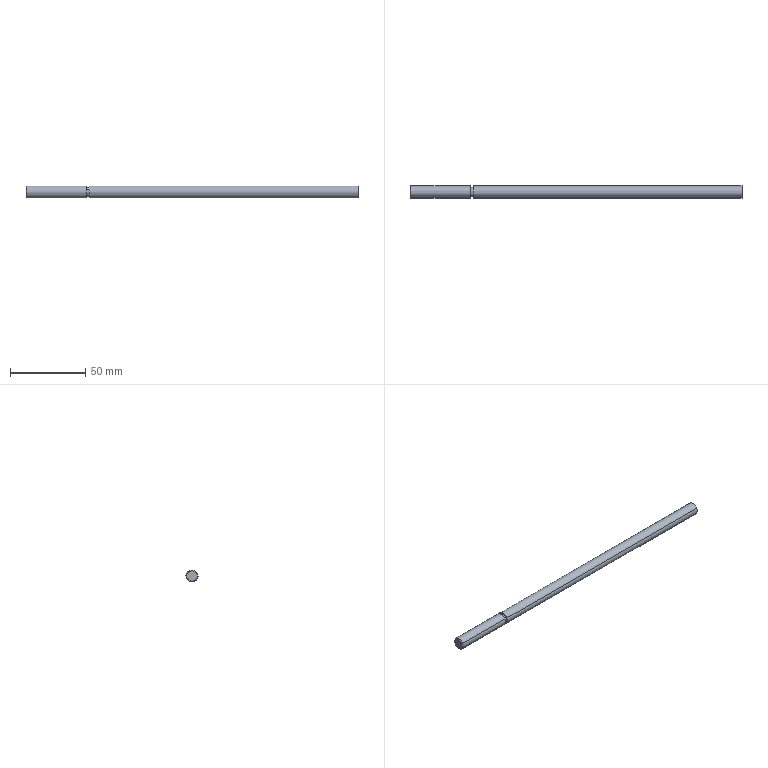Component | SolidWorks | 007GuideRod-2 | 1 solid | 16 faces | box 220 x 8 x 8 mm | volume 10834 mm3 | cylinder 8 | cone 4 | plane 4 | commonest cylinder face diameters 8 x4 6 x2 4.2 x2
build123d program:
from build123d import *

# Parameters (mm, degrees)
SKETCH1_R                 = 4
EXTRUDE1_DEPTH            = 110
M5X0_8_TAPPED_HOLE1_D     = 4.2
M5X0_8_TAPPED_HOLE1_DEPTH = 12.4
M5X0_8_TAPPED_HOLE1_TIP   = 1.262
CHAMFER1_SIZE             = 0.5
SKETCH4_W                 = 1
SKETCH4_H                 = 2


with BuildPart() as part:
    # Sketch1 → Extrude1 (new, symmetric)
    with BuildSketch(Plane.XY):
        Circle(SKETCH1_R)
    extrude(amount=EXTRUDE1_DEPTH, both=True)

    # M5x0.8 Tapped Hole1
    with Locations(Plane.XY.offset(110)):
        with Locations((0, 0)):
            Hole(M5X0_8_TAPPED_HOLE1_D / 2, depth=M5X0_8_TAPPED_HOLE1_DEPTH)
            with Locations((0, 0, -(M5X0_8_TAPPED_HOLE1_DEPTH + M5X0_8_TAPPED_HOLE1_TIP / 2))):  # 118° drill point
                Cone(0, M5X0_8_TAPPED_HOLE1_D / 2, M5X0_8_TAPPED_HOLE1_TIP, mode=Mode.SUBTRACT)

    # Chamfer1
    chamfer1_edges = [part.edges().sort_by_distance(p)[0] for p in [
        (-4, 0, -110),
    ]]
    chamfer(chamfer1_edges, length=CHAMFER1_SIZE)

    # Sketch4 → Cut-Revolve1 (revolve, cut)
    with BuildSketch(Plane(origin=(0, 0, 0), x_dir=(1, 0, 0), z_dir=(0, 1, 0))):
        with Locations((-3.5, 69)):
            Rectangle(SKETCH4_W, SKETCH4_H)
    revolve(axis=Axis((0, 0, -71.443), (0, 0, 1)), mode=Mode.SUBTRACT)


solid = part.part

# Placed as in the assembly
solid = solid.moved(Location((-83.24, 24.924, 53.04), (0, 90, 0)))
STEP:
#1=CARTESIAN_POINT('',(-6.033,1.121,2.016));
#2=VERTEX_POINT('',#1);
#3=CARTESIAN_POINT('',(-6.033,0.8413,2.16));
#4=VERTEX_POINT('',#3);
#5=CARTESIAN_POINT('',(-6.033,0.9813,2.088));
#6=DIRECTION('',(-1.,-0.,0.));
#7=DIRECTION('',(0.,0.8889,-0.4581));
#8=AXIS2_PLACEMENT_3D('',#5,#6,#7);
#9=CIRCLE('',#8,0.1575);
#10=EDGE_CURVE('',#2,#4,#9,.T.);
#11=ORIENTED_EDGE('',*,*,#10,.T.);
#12=CARTESIAN_POINT('',(-7.588,0.8413,2.16));
#13=VERTEX_POINT('',#12);
#14=CARTESIAN_POINT('',(1.054,0.8413,2.16));
#15=DIRECTION('',(-1.,-0.,0.));
#16=VECTOR('',#15,39.37);
#17=LINE('',#14,#16);
#18=EDGE_CURVE('',#4,#13,#17,.T.);
#19=ORIENTED_EDGE('',*,*,#18,.T.);
#20=CARTESIAN_POINT('',(-7.588,1.121,2.016));
#21=VERTEX_POINT('',#20);
#22=CARTESIAN_POINT('',(-7.588,0.9813,2.088));
#23=DIRECTION('',(1.,0.,-0.));
#24=DIRECTION('',(0.,-0.8889,0.4581));
#25=AXIS2_PLACEMENT_3D('',#22,#23,#24);
#26=CIRCLE('',#25,0.1575);
#27=EDGE_CURVE('',#13,#21,#26,.T.);
#28=ORIENTED_EDGE('',*,*,#27,.T.);
#29=CARTESIAN_POINT('',(1.054,1.121,2.016));
#30=DIRECTION('',(-1.,-0.,0.));
#31=VECTOR('',#30,39.37);
#32=LINE('',#29,#31);
#33=EDGE_CURVE('',#2,#21,#32,.T.);
#34=ORIENTED_EDGE('',*,*,#33,.F.);
#35=EDGE_LOOP('',(#11,#19,#28,#34));
#36=FACE_OUTER_BOUND('',#35,.T.);
#37=CARTESIAN_POINT('',(1.054,0.9813,2.088));
#38=DIRECTION('',(-1.,-0.,0.));
#39=DIRECTION('',(0.,0.8889,-0.4581));
#40=AXIS2_PLACEMENT_3D('',#37,#38,#39);
#41=CYLINDRICAL_SURFACE('',#40,0.1575);
#42=ADVANCED_FACE('',(#36),#41,.T.);
#43=CARTESIAN_POINT('',(-7.608,1.104,2.025));
#44=VERTEX_POINT('',#43);
#45=CARTESIAN_POINT('',(-7.608,0.8588,2.151));
#46=VERTEX_POINT('',#45);
#47=CARTESIAN_POINT('',(-7.608,0.9813,2.088));
#48=DIRECTION('',(-1.,-0.,0.));
#49=DIRECTION('',(0.,-0.8889,0.4581));
#50=AXIS2_PLACEMENT_3D('',#47,#48,#49);
#51=CIRCLE('',#50,0.1378);
#52=EDGE_CURVE('',#44,#46,#51,.T.);
#53=ORIENTED_EDGE('',*,*,#52,.F.);
#54=CARTESIAN_POINT('',(-7.588,1.121,2.016));
#55=DIRECTION('',(0.7071,0.6285,-0.3239));
#56=VECTOR('',#55,39.37);
#57=LINE('',#54,#56);
#58=EDGE_CURVE('',#44,#21,#57,.T.);
#59=ORIENTED_EDGE('',*,*,#58,.T.);
#60=ORIENTED_EDGE('',*,*,#27,.F.);
#61=CARTESIAN_POINT('',(-7.588,0.8413,2.16));
#62=DIRECTION('',(0.7071,-0.6285,0.3239));
#63=VECTOR('',#62,39.37);
#64=LINE('',#61,#63);
#65=EDGE_CURVE('',#46,#13,#64,.T.);
#66=ORIENTED_EDGE('',*,*,#65,.F.);
#67=EDGE_LOOP('',(#53,#59,#60,#66));
#68=FACE_OUTER_BOUND('',#67,.T.);
#69=CARTESIAN_POINT('',(-7.588,0.9813,2.088));
#70=DIRECTION('',(1.,0.,-0.));
#71=DIRECTION('',(0.,-0.8889,0.4581));
#72=AXIS2_PLACEMENT_3D('',#69,#70,#71);
#73=CONICAL_SURFACE('',#72,0.1575,0.7854);
#74=ADVANCED_FACE('',(#68),#73,.T.);
#75=CARTESIAN_POINT('',(-5.954,1.086,2.034));
#76=VERTEX_POINT('',#75);
#77=CARTESIAN_POINT('',(-5.954,0.8763,2.142));
#78=VERTEX_POINT('',#77);
#79=CARTESIAN_POINT('',(-5.954,0.9813,2.088));
#80=DIRECTION('',(-1.,-0.,0.));
#81=DIRECTION('',(0.,0.8889,-0.4581));
#82=AXIS2_PLACEMENT_3D('',#79,#80,#81);
#83=CIRCLE('',#82,0.1181);
#84=EDGE_CURVE('',#76,#78,#83,.T.);
#85=ORIENTED_EDGE('',*,*,#84,.T.);
#86=CARTESIAN_POINT('',(-6.033,0.8763,2.142));
#87=VERTEX_POINT('',#86);
#88=CARTESIAN_POINT('',(-6.09,0.8763,2.142));
#89=DIRECTION('',(-1.,-0.,0.));
#90=VECTOR('',#89,39.37);
#91=LINE('',#88,#90);
#92=EDGE_CURVE('',#78,#87,#91,.T.);
#93=ORIENTED_EDGE('',*,*,#92,.T.);
#94=CARTESIAN_POINT('',(-6.033,1.086,2.034));
#95=VERTEX_POINT('',#94);
#96=CARTESIAN_POINT('',(-6.033,0.9813,2.088));
#97=DIRECTION('',(-1.,-0.,0.));
#98=DIRECTION('',(0.,0.8889,-0.4581));
#99=AXIS2_PLACEMENT_3D('',#96,#97,#98);
#100=CIRCLE('',#99,0.1181);
#101=EDGE_CURVE('',#95,#87,#100,.T.);
#102=ORIENTED_EDGE('',*,*,#101,.F.);
#103=CARTESIAN_POINT('',(-6.09,1.086,2.034));
#104=DIRECTION('',(-1.,-0.,0.));
#105=VECTOR('',#104,39.37);
#106=LINE('',#103,#105);
#107=EDGE_CURVE('',#76,#95,#106,.T.);
#108=ORIENTED_EDGE('',*,*,#107,.F.);
#109=EDGE_LOOP('',(#85,#93,#102,#108));
#110=FACE_OUTER_BOUND('',#109,.T.);
#111=CARTESIAN_POINT('',(-6.09,0.9813,2.088));
#112=DIRECTION('',(-1.,-0.,0.));
#113=DIRECTION('',(0.,0.8889,-0.4581));
#114=AXIS2_PLACEMENT_3D('',#111,#112,#113);
#115=CYLINDRICAL_SURFACE('',#114,0.1181);
#116=ADVANCED_FACE('',(#110),#115,.T.);
#117=CARTESIAN_POINT('',(0.5157,0.9813,2.088));
#118=VERTEX_POINT('',#117);
#119=CARTESIAN_POINT('',(0.5653,0.9078,2.126));
#120=VERTEX_POINT('',#119);
#121=CARTESIAN_POINT('',(0.5653,0.9078,2.126));
#122=DIRECTION('',(0.515,-0.7619,0.3927));
#123=VECTOR('',#122,39.37);
#124=LINE('',#121,#123);
#125=EDGE_CURVE('',#118,#120,#124,.T.);
#126=ORIENTED_EDGE('',*,*,#125,.F.);
#127=CARTESIAN_POINT('',(0.5653,1.055,2.05));
#128=VERTEX_POINT('',#127);
#129=CARTESIAN_POINT('',(0.5653,1.055,2.05));
#130=DIRECTION('',(0.515,0.7619,-0.3927));
#131=VECTOR('',#130,39.37);
#132=LINE('',#129,#131);
#133=EDGE_CURVE('',#118,#128,#132,.T.);
#134=ORIENTED_EDGE('',*,*,#133,.T.);
#135=CARTESIAN_POINT('',(0.5653,0.9813,2.088));
#136=DIRECTION('',(1.,0.,-0.));
#137=DIRECTION('',(0.,-0.8889,0.4581));
#138=AXIS2_PLACEMENT_3D('',#135,#136,#137);
#139=CIRCLE('',#138,0.08268);
#140=EDGE_CURVE('',#128,#120,#139,.T.);
#141=ORIENTED_EDGE('',*,*,#140,.T.);
#142=EDGE_LOOP('',(#126,#134,#141));
#143=FACE_OUTER_BOUND('',#142,.T.);
#144=CARTESIAN_POINT('',(0.5653,0.9813,2.088));
#145=DIRECTION('',(1.,0.,-0.));
#146=DIRECTION('',(0.,-0.8889,0.4581));
#147=AXIS2_PLACEMENT_3D('',#144,#145,#146);
#148=CONICAL_SURFACE('',#147,0.08268,1.03);
#149=ADVANCED_FACE('',(#143),#148,.F.);
#150=ORIENTED_EDGE('',*,*,#140,.F.);
#151=CARTESIAN_POINT('',(1.054,1.055,2.05));
#152=VERTEX_POINT('',#151);
#153=CARTESIAN_POINT('',(1.054,1.055,2.05));
#154=DIRECTION('',(1.,0.,-0.));
#155=VECTOR('',#154,39.37);
#156=LINE('',#153,#155);
#157=EDGE_CURVE('',#128,#152,#156,.T.);
#158=ORIENTED_EDGE('',*,*,#157,.T.);
#159=CARTESIAN_POINT('',(1.054,0.9078,2.126));
#160=VERTEX_POINT('',#159);
#161=CARTESIAN_POINT('',(1.054,0.9813,2.088));
#162=DIRECTION('',(1.,0.,-0.));
#163=DIRECTION('',(0.,-0.8889,0.4581));
#164=AXIS2_PLACEMENT_3D('',#161,#162,#163);
#165=CIRCLE('',#164,0.08268);
#166=EDGE_CURVE('',#152,#160,#165,.T.);
#167=ORIENTED_EDGE('',*,*,#166,.T.);
#168=CARTESIAN_POINT('',(1.054,0.9078,2.126));
#169=DIRECTION('',(1.,0.,-0.));
#170=VECTOR('',#169,39.37);
#171=LINE('',#168,#170);
#172=EDGE_CURVE('',#120,#160,#171,.T.);
#173=ORIENTED_EDGE('',*,*,#172,.F.);
#174=EDGE_LOOP('',(#150,#158,#167,#173));
#175=FACE_OUTER_BOUND('',#174,.T.);
#176=CARTESIAN_POINT('',(1.054,0.9813,2.088));
#177=DIRECTION('',(1.,0.,-0.));
#178=DIRECTION('',(0.,-0.8889,0.4581));
#179=AXIS2_PLACEMENT_3D('',#176,#177,#178);
#180=CYLINDRICAL_SURFACE('',#179,0.08268);
#181=ADVANCED_FACE('',(#175),#180,.F.);
#182=CARTESIAN_POINT('',(1.054,0.8413,2.16));
#183=VERTEX_POINT('',#182);
#184=CARTESIAN_POINT('',(1.054,1.121,2.016));
#185=VERTEX_POINT('',#184);
#186=CARTESIAN_POINT('',(1.054,0.9813,2.088));
#187=DIRECTION('',(1.,0.,-0.));
#188=DIRECTION('',(0.,-0.8889,0.4581));
#189=AXIS2_PLACEMENT_3D('',#186,#187,#188);
#190=CIRCLE('',#189,0.1575);
#191=EDGE_CURVE('',#183,#185,#190,.T.);
#192=ORIENTED_EDGE('',*,*,#191,.F.);
#193=CARTESIAN_POINT('',(-5.954,0.8413,2.16));
#194=VERTEX_POINT('',#193);
#195=CARTESIAN_POINT('',(1.054,0.8413,2.16));
#196=DIRECTION('',(-1.,-0.,0.));
#197=VECTOR('',#196,39.37);
#198=LINE('',#195,#197);
#199=EDGE_CURVE('',#183,#194,#198,.T.);
#200=ORIENTED_EDGE('',*,*,#199,.T.);
#201=CARTESIAN_POINT('',(-5.954,1.121,2.016));
#202=VERTEX_POINT('',#201);
#203=CARTESIAN_POINT('',(-5.954,0.9813,2.088));
#204=DIRECTION('',(-1.,-0.,0.));
#205=DIRECTION('',(0.,0.8889,-0.4581));
#206=AXIS2_PLACEMENT_3D('',#203,#204,#205);
#207=CIRCLE('',#206,0.1575);
#208=EDGE_CURVE('',#202,#194,#207,.T.);
#209=ORIENTED_EDGE('',*,*,#208,.F.);
#210=CARTESIAN_POINT('',(1.054,1.121,2.016));
#211=DIRECTION('',(-1.,-0.,0.));
#212=VECTOR('',#211,39.37);
#213=LINE('',#210,#212);
#214=EDGE_CURVE('',#185,#202,#213,.T.);
#215=ORIENTED_EDGE('',*,*,#214,.F.);
#216=EDGE_LOOP('',(#192,#200,#209,#215));
#217=FACE_OUTER_BOUND('',#216,.T.);
#218=CARTESIAN_POINT('',(1.054,0.9813,2.088));
#219=DIRECTION('',(-1.,-0.,0.));
#220=DIRECTION('',(0.,0.8889,-0.4581));
#221=AXIS2_PLACEMENT_3D('',#218,#219,#220);
#222=CYLINDRICAL_SURFACE('',#221,0.1575);
#223=ADVANCED_FACE('',(#217),#222,.T.);
#224=ORIENTED_EDGE('',*,*,#199,.F.);
#225=CARTESIAN_POINT('',(1.054,0.9813,2.088));
#226=DIRECTION('',(1.,0.,-0.));
#227=DIRECTION('',(0.,-0.8889,0.4581));
#228=AXIS2_PLACEMENT_3D('',#225,#226,#227);
#229=CIRCLE('',#228,0.1575);
#230=EDGE_CURVE('',#185,#183,#229,.T.);
#231=ORIENTED_EDGE('',*,*,#230,.F.);
#232=ORIENTED_EDGE('',*,*,#214,.T.);
#233=CARTESIAN_POINT('',(-5.954,0.9813,2.088));
#234=DIRECTION('',(-1.,-0.,0.));
#235=DIRECTION('',(0.,0.8889,-0.4581));
#236=AXIS2_PLACEMENT_3D('',#233,#234,#235);
#237=CIRCLE('',#236,0.1575);
#238=EDGE_CURVE('',#194,#202,#237,.T.);
#239=ORIENTED_EDGE('',*,*,#238,.F.);
#240=EDGE_LOOP('',(#224,#231,#232,#239));
#241=FACE_OUTER_BOUND('',#240,.T.);
#242=CARTESIAN_POINT('',(1.054,0.9813,2.088));
#243=DIRECTION('',(-1.,-0.,0.));
#244=DIRECTION('',(0.,0.8889,-0.4581));
#245=AXIS2_PLACEMENT_3D('',#242,#243,#244);
#246=CYLINDRICAL_SURFACE('',#245,0.1575);
#247=ADVANCED_FACE('',(#241),#246,.T.);
#248=CARTESIAN_POINT('',(1.054,0.9813,2.088));
#249=DIRECTION('',(1.,0.,-0.));
#250=DIRECTION('',(0.,-0.8889,0.4581));
#251=AXIS2_PLACEMENT_3D('',#248,#249,#250);
#252=CIRCLE('',#251,0.08268);
#253=EDGE_CURVE('',#160,#152,#252,.T.);
#254=ORIENTED_EDGE('',*,*,#253,.F.);
#255=ORIENTED_EDGE('',*,*,#166,.F.);
#256=EDGE_LOOP('',(#254,#255));
#257=FACE_BOUND('',#256,.T.);
#258=ORIENTED_EDGE('',*,*,#230,.T.);
#259=ORIENTED_EDGE('',*,*,#191,.T.);
#260=EDGE_LOOP('',(#258,#259));
#261=FACE_OUTER_BOUND('',#260,.T.);
#262=CARTESIAN_POINT('',(1.054,0.9813,2.088));
#263=DIRECTION('',(1.,0.,-0.));
#264=DIRECTION('',(0.,-0.8889,0.4581));
#265=AXIS2_PLACEMENT_3D('',#262,#263,#264);
#266=PLANE('',#265);
#267=ADVANCED_FACE('',(#257,#261),#266,.T.);
#268=ORIENTED_EDGE('',*,*,#157,.F.);
#269=CARTESIAN_POINT('',(0.5653,0.9813,2.088));
#270=DIRECTION('',(1.,0.,-0.));
#271=DIRECTION('',(0.,-0.8889,0.4581));
#272=AXIS2_PLACEMENT_3D('',#269,#270,#271);
#273=CIRCLE('',#272,0.08268);
#274=EDGE_CURVE('',#120,#128,#273,.T.);
#275=ORIENTED_EDGE('',*,*,#274,.F.);
#276=ORIENTED_EDGE('',*,*,#172,.T.);
#277=ORIENTED_EDGE('',*,*,#253,.T.);
#278=EDGE_LOOP('',(#268,#275,#276,#277));
#279=FACE_OUTER_BOUND('',#278,.T.);
#280=CARTESIAN_POINT('',(1.054,0.9813,2.088));
#281=DIRECTION('',(1.,0.,-0.));
#282=DIRECTION('',(0.,-0.8889,0.4581));
#283=AXIS2_PLACEMENT_3D('',#280,#281,#282);
#284=CYLINDRICAL_SURFACE('',#283,0.08268);
#285=ADVANCED_FACE('',(#279),#284,.F.);
#286=ORIENTED_EDGE('',*,*,#133,.F.);
#287=ORIENTED_EDGE('',*,*,#125,.T.);
#288=ORIENTED_EDGE('',*,*,#274,.T.);
#289=EDGE_LOOP('',(#286,#287,#288));
#290=FACE_OUTER_BOUND('',#289,.T.);
#291=CARTESIAN_POINT('',(0.5653,0.9813,2.088));
#292=DIRECTION('',(1.,0.,-0.));
#293=DIRECTION('',(0.,-0.8889,0.4581));
#294=AXIS2_PLACEMENT_3D('',#291,#292,#293);
#295=CONICAL_SURFACE('',#294,0.08268,1.03);
#296=ADVANCED_FACE('',(#290),#295,.F.);
#297=ORIENTED_EDGE('',*,*,#10,.F.);
#298=CARTESIAN_POINT('',(-6.033,0.9813,2.088));
#299=DIRECTION('',(-1.,-0.,0.));
#300=DIRECTION('',(0.,0.8889,-0.4581));
#301=AXIS2_PLACEMENT_3D('',#298,#299,#300);
#302=CIRCLE('',#301,0.1575);
#303=EDGE_CURVE('',#4,#2,#302,.T.);
#304=ORIENTED_EDGE('',*,*,#303,.F.);
#305=EDGE_LOOP('',(#297,#304));
#306=FACE_OUTER_BOUND('',#305,.T.);
#307=ORIENTED_EDGE('',*,*,#101,.T.);
#308=CARTESIAN_POINT('',(-6.033,0.9813,2.088));
#309=DIRECTION('',(-1.,-0.,0.));
#310=DIRECTION('',(0.,0.8889,-0.4581));
#311=AXIS2_PLACEMENT_3D('',#308,#309,#310);
#312=CIRCLE('',#311,0.1181);
#313=EDGE_CURVE('',#87,#95,#312,.T.);
#314=ORIENTED_EDGE('',*,*,#313,.T.);
#315=EDGE_LOOP('',(#307,#314));
#316=FACE_BOUND('',#315,.T.);
#317=CARTESIAN_POINT('',(-6.033,1.121,2.016));
#318=DIRECTION('',(-1.,-0.,0.));
#319=DIRECTION('',(-0.,0.8889,-0.4581));
#320=AXIS2_PLACEMENT_3D('',#317,#318,#319);
#321=PLANE('',#320);
#322=ADVANCED_FACE('',(#306,#316),#321,.F.);
#323=ORIENTED_EDGE('',*,*,#92,.F.);
#324=CARTESIAN_POINT('',(-5.954,0.9813,2.088));
#325=DIRECTION('',(-1.,-0.,0.));
#326=DIRECTION('',(0.,0.8889,-0.4581));
#327=AXIS2_PLACEMENT_3D('',#324,#325,#326);
#328=CIRCLE('',#327,0.1181);
#329=EDGE_CURVE('',#78,#76,#328,.T.);
#330=ORIENTED_EDGE('',*,*,#329,.T.);
#331=ORIENTED_EDGE('',*,*,#107,.T.);
#332=ORIENTED_EDGE('',*,*,#313,.F.);
#333=EDGE_LOOP('',(#323,#330,#331,#332));
#334=FACE_OUTER_BOUND('',#333,.T.);
#335=CARTESIAN_POINT('',(-6.09,0.9813,2.088));
#336=DIRECTION('',(-1.,-0.,0.));
#337=DIRECTION('',(0.,0.8889,-0.4581));
#338=AXIS2_PLACEMENT_3D('',#335,#336,#337);
#339=CYLINDRICAL_SURFACE('',#338,0.1181);
#340=ADVANCED_FACE('',(#334),#339,.T.);
#341=ORIENTED_EDGE('',*,*,#84,.F.);
#342=ORIENTED_EDGE('',*,*,#329,.F.);
#343=EDGE_LOOP('',(#341,#342));
#344=FACE_BOUND('',#343,.T.);
#345=ORIENTED_EDGE('',*,*,#208,.T.);
#346=ORIENTED_EDGE('',*,*,#238,.T.);
#347=EDGE_LOOP('',(#345,#346));
#348=FACE_OUTER_BOUND('',#347,.T.);
#349=CARTESIAN_POINT('',(-5.954,1.086,2.034));
#350=DIRECTION('',(1.,0.,-0.));
#351=DIRECTION('',(0.,-0.8889,0.4581));
#352=AXIS2_PLACEMENT_3D('',#349,#350,#351);
#353=PLANE('',#352);
#354=ADVANCED_FACE('',(#344,#348),#353,.F.);
#355=CARTESIAN_POINT('',(-7.608,0.9813,2.088));
#356=DIRECTION('',(-1.,-0.,0.));
#357=DIRECTION('',(0.,-0.8889,0.4581));
#358=AXIS2_PLACEMENT_3D('',#355,#356,#357);
#359=CIRCLE('',#358,0.1378);
#360=EDGE_CURVE('',#46,#44,#359,.T.);
#361=ORIENTED_EDGE('',*,*,#360,.T.);
#362=ORIENTED_EDGE('',*,*,#52,.T.);
#363=EDGE_LOOP('',(#361,#362));
#364=FACE_OUTER_BOUND('',#363,.T.);
#365=CARTESIAN_POINT('',(-7.608,0.9813,2.088));
#366=DIRECTION('',(1.,0.,-0.));
#367=DIRECTION('',(0.,-0.8889,0.4581));
#368=AXIS2_PLACEMENT_3D('',#365,#366,#367);
#369=PLANE('',#368);
#370=ADVANCED_FACE('',(#364),#369,.F.);
#371=ORIENTED_EDGE('',*,*,#58,.F.);
#372=ORIENTED_EDGE('',*,*,#360,.F.);
#373=ORIENTED_EDGE('',*,*,#65,.T.);
#374=CARTESIAN_POINT('',(-7.588,0.9813,2.088));
#375=DIRECTION('',(1.,0.,-0.));
#376=DIRECTION('',(0.,-0.8889,0.4581));
#377=AXIS2_PLACEMENT_3D('',#374,#375,#376);
#378=CIRCLE('',#377,0.1575);
#379=EDGE_CURVE('',#21,#13,#378,.T.);
#380=ORIENTED_EDGE('',*,*,#379,.F.);
#381=EDGE_LOOP('',(#371,#372,#373,#380));
#382=FACE_OUTER_BOUND('',#381,.T.);
#383=CARTESIAN_POINT('',(-7.588,0.9813,2.088));
#384=DIRECTION('',(1.,0.,-0.));
#385=DIRECTION('',(0.,-0.8889,0.4581));
#386=AXIS2_PLACEMENT_3D('',#383,#384,#385);
#387=CONICAL_SURFACE('',#386,0.1575,0.7854);
#388=ADVANCED_FACE('',(#382),#387,.T.);
#389=ORIENTED_EDGE('',*,*,#18,.F.);
#390=ORIENTED_EDGE('',*,*,#303,.T.);
#391=ORIENTED_EDGE('',*,*,#33,.T.);
#392=ORIENTED_EDGE('',*,*,#379,.T.);
#393=EDGE_LOOP('',(#389,#390,#391,#392));
#394=FACE_OUTER_BOUND('',#393,.T.);
#395=CARTESIAN_POINT('',(1.054,0.9813,2.088));
#396=DIRECTION('',(-1.,-0.,0.));
#397=DIRECTION('',(0.,0.8889,-0.4581));
#398=AXIS2_PLACEMENT_3D('',#395,#396,#397);
#399=CYLINDRICAL_SURFACE('',#398,0.1575);
#400=ADVANCED_FACE('',(#394),#399,.T.);
#401=CLOSED_SHELL('',(#42,#74,#116,#149,#181,#223,#247,#267,#285,#296,#322,#340,#354,#370,#388,#400));
#402=MANIFOLD_SOLID_BREP('',#401);
#403=CARTESIAN_POINT('',(0.,0.,0.));
#404=DIRECTION('',(0.,0.,1.));
#405=DIRECTION('',(1.,0.,0.));
#406=AXIS2_PLACEMENT_3D('',#403,#404,#405);
#407=(LENGTH_UNIT()NAMED_UNIT(*)SI_UNIT($,.METRE.));
#408=LENGTH_MEASURE_WITH_UNIT(LENGTH_MEASURE(0.0254),#407);
#409=DIMENSIONAL_EXPONENTS(1.,0.,0.,0.,0.,0.,0.);
#410=(CONVERSION_BASED_UNIT('',#408)LENGTH_UNIT()NAMED_UNIT(#409));
#411=UNCERTAINTY_MEASURE_WITH_UNIT(LENGTH_MEASURE(0.00001),#410,'','');
#412=(NAMED_UNIT(*)PLANE_ANGLE_UNIT()SI_UNIT($,.RADIAN.));
#413=(NAMED_UNIT(*)SI_UNIT($,.STERADIAN.)SOLID_ANGLE_UNIT());
#414=(GEOMETRIC_REPRESENTATION_CONTEXT(3)GLOBAL_UNCERTAINTY_ASSIGNED_CONTEXT((#411))GLOBAL_UNIT_ASSIGNED_CONTEXT((#410,#412,#413))REPRESENTATION_CONTEXT('',''));
#415=ADVANCED_BREP_SHAPE_REPRESENTATION('',(#402,#406),#414);
#416=COLOUR_RGB('',0.7922,0.8196,0.9333);
#417=FILL_AREA_STYLE_COLOUR('',#416);
#418=FILL_AREA_STYLE('',(#417));
#419=SURFACE_STYLE_FILL_AREA(#418);
#420=SURFACE_SIDE_STYLE('',(#419));
#421=SURFACE_STYLE_USAGE(.BOTH.,#420);
#422=PRESENTATION_STYLE_ASSIGNMENT((#421));
#423=STYLED_ITEM('',(#422),#402);
#424=PRESENTATION_LAYER_ASSIGNMENT('','',(#423));
#425=(LENGTH_UNIT()NAMED_UNIT(*)SI_UNIT($,.METRE.));
#426=LENGTH_MEASURE_WITH_UNIT(LENGTH_MEASURE(0.0254),#425);
#427=DIMENSIONAL_EXPONENTS(1.,0.,0.,0.,0.,0.,0.);
#428=(CONVERSION_BASED_UNIT('',#426)LENGTH_UNIT()NAMED_UNIT(#427));
#429=UNCERTAINTY_MEASURE_WITH_UNIT(LENGTH_MEASURE(0.00001),#428,'','');
#430=(NAMED_UNIT(*)PLANE_ANGLE_UNIT()SI_UNIT($,.RADIAN.));
#431=(NAMED_UNIT(*)SI_UNIT($,.STERADIAN.)SOLID_ANGLE_UNIT());
#432=(GEOMETRIC_REPRESENTATION_CONTEXT(3)GLOBAL_UNCERTAINTY_ASSIGNED_CONTEXT((#429))GLOBAL_UNIT_ASSIGNED_CONTEXT((#428,#430,#431))REPRESENTATION_CONTEXT('',''));
#433=MECHANICAL_DESIGN_GEOMETRIC_PRESENTATION_REPRESENTATION('',(#423),#432);